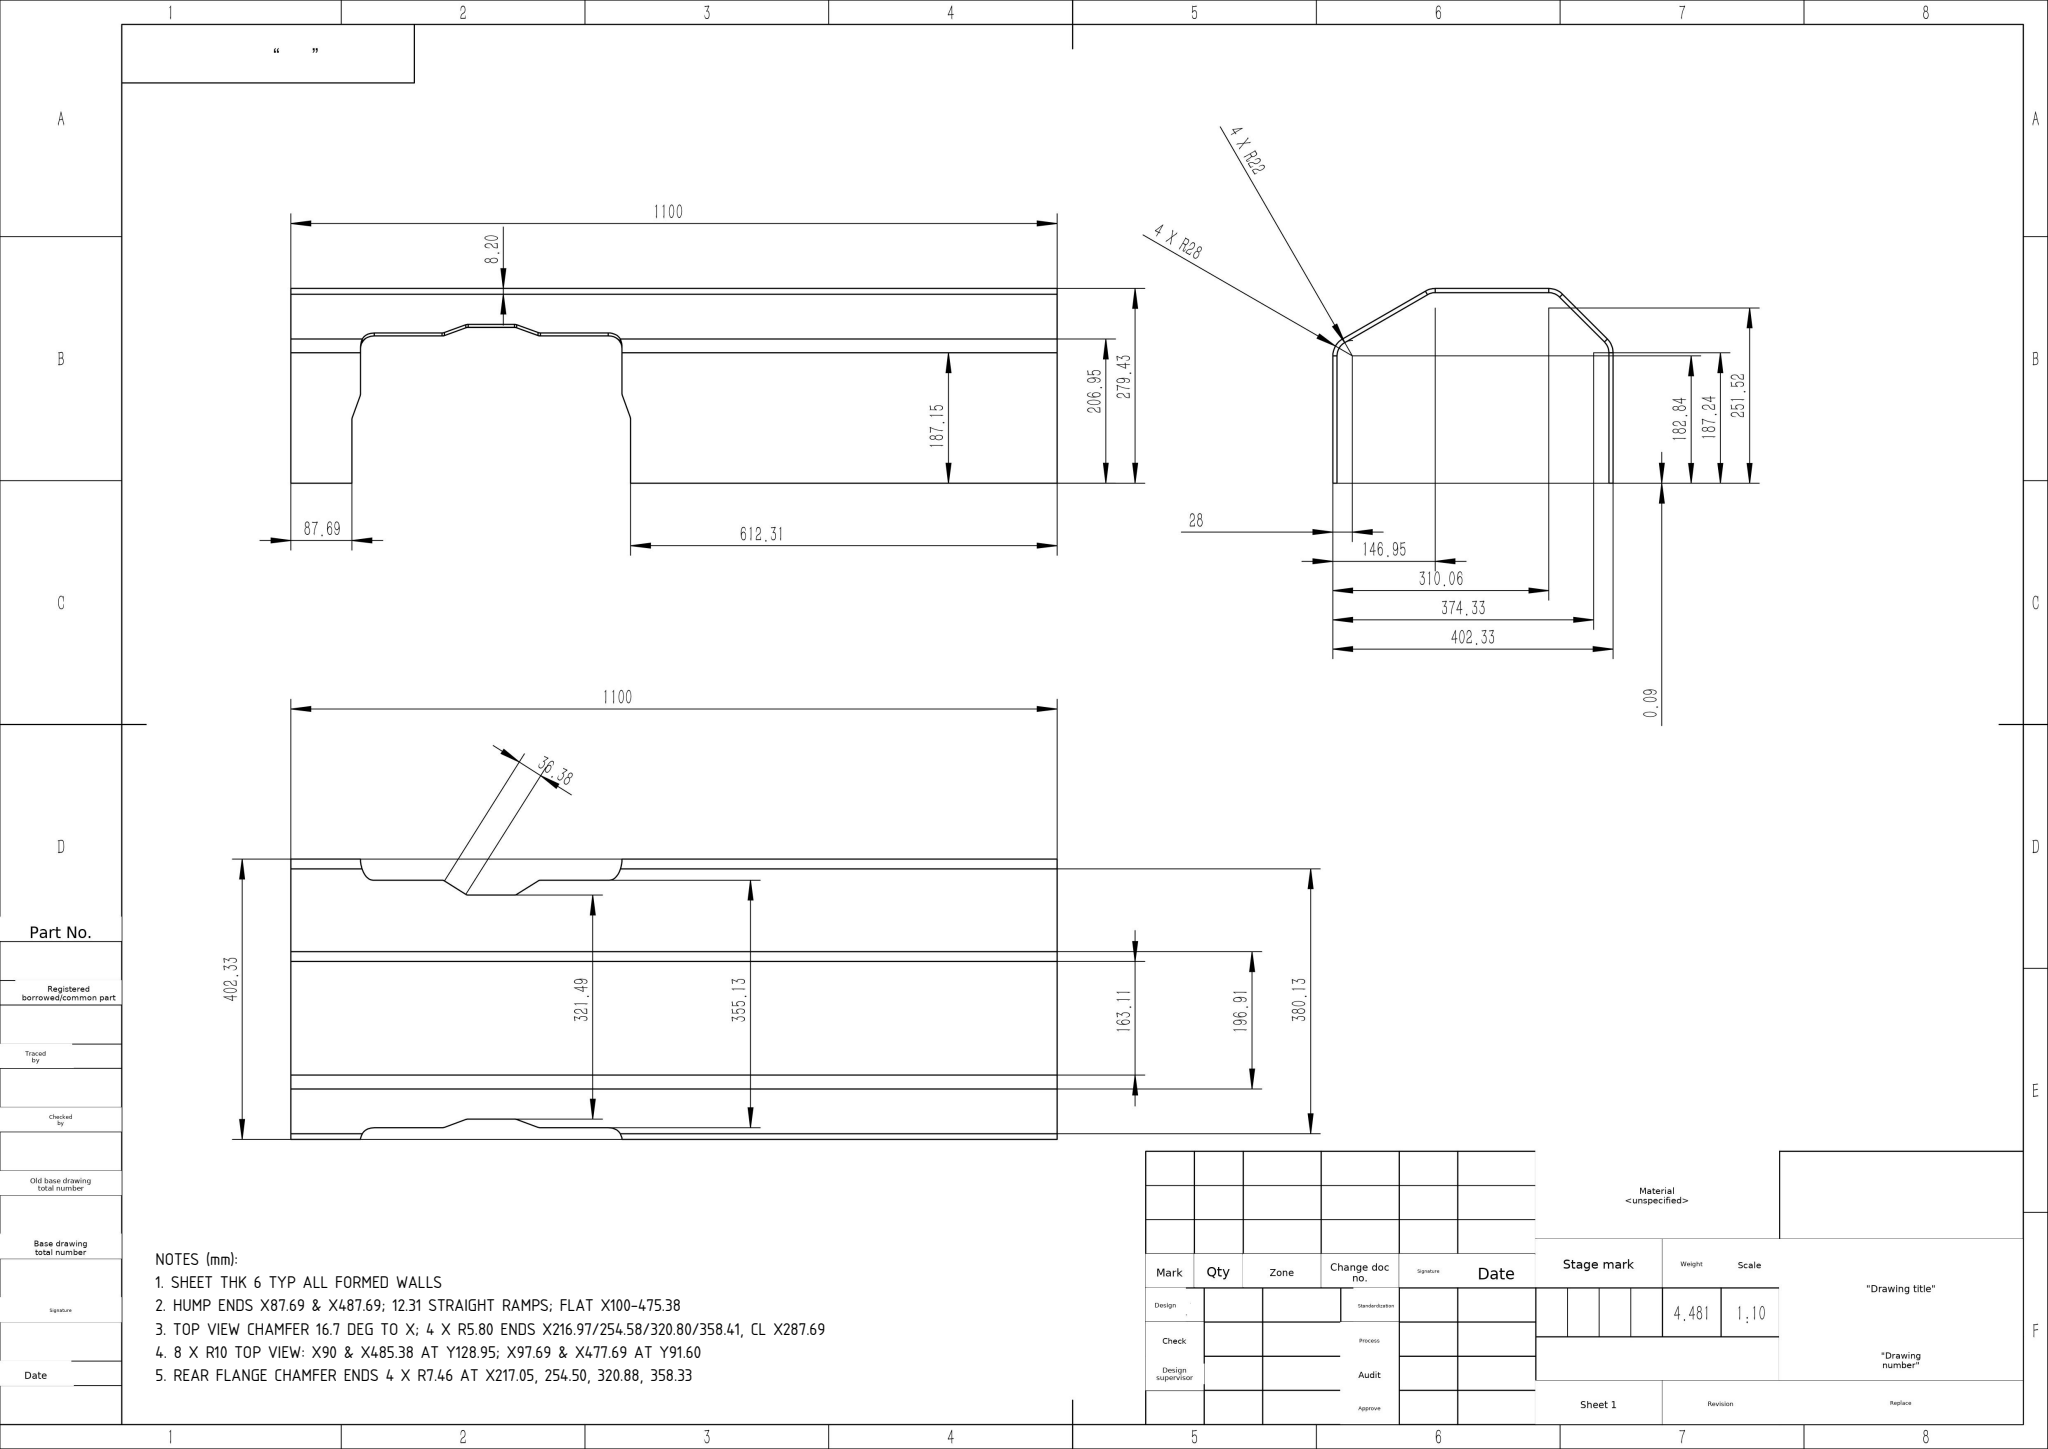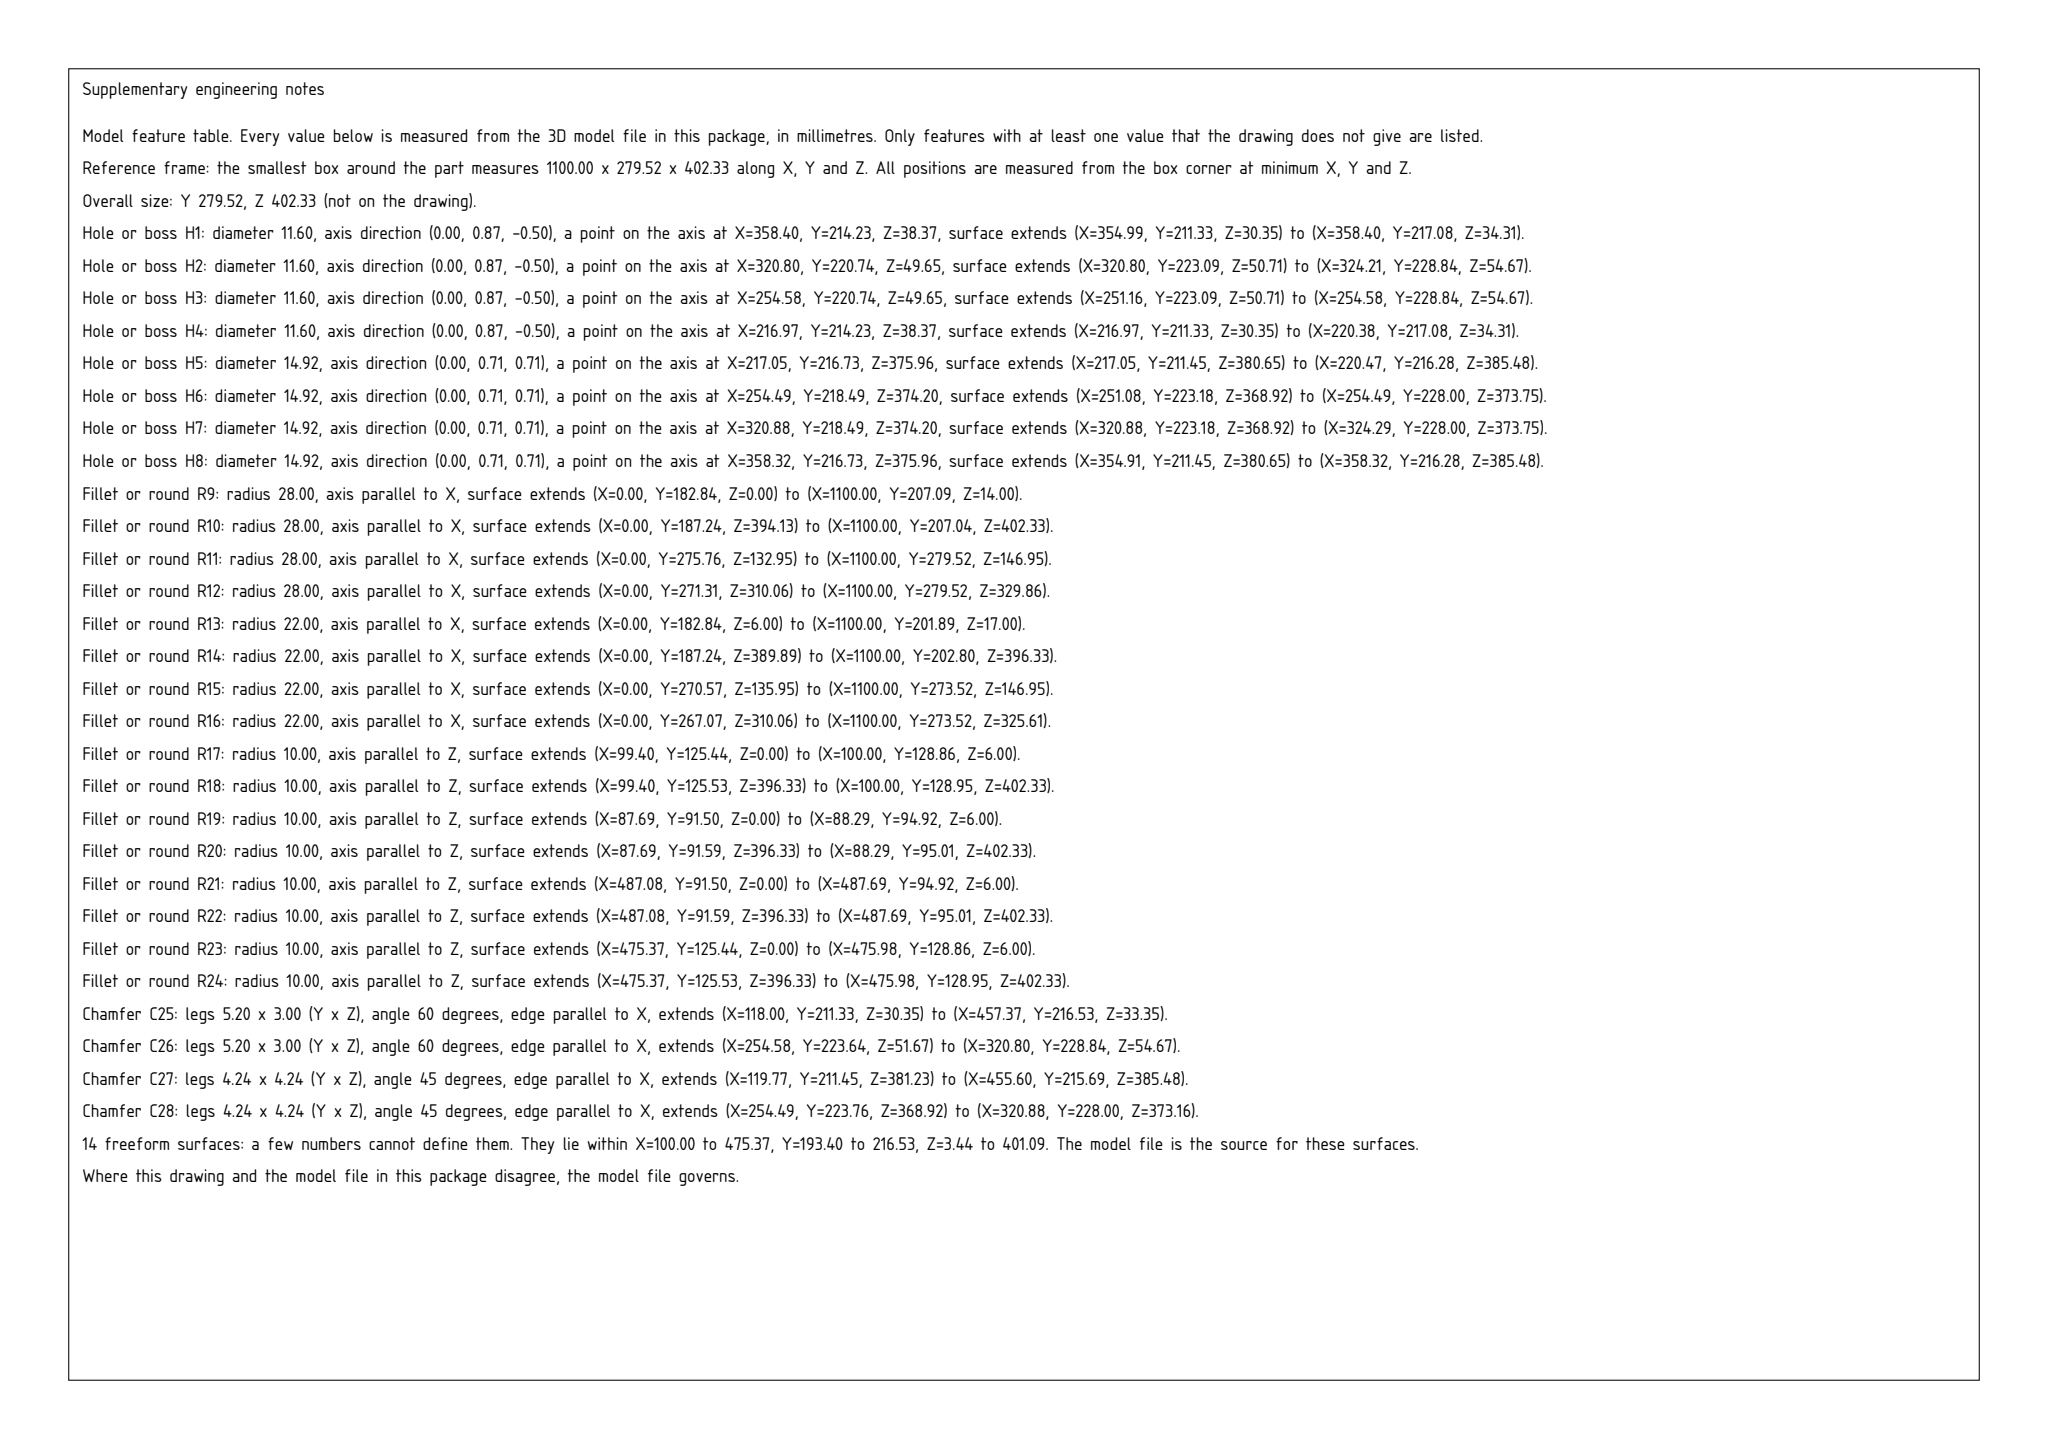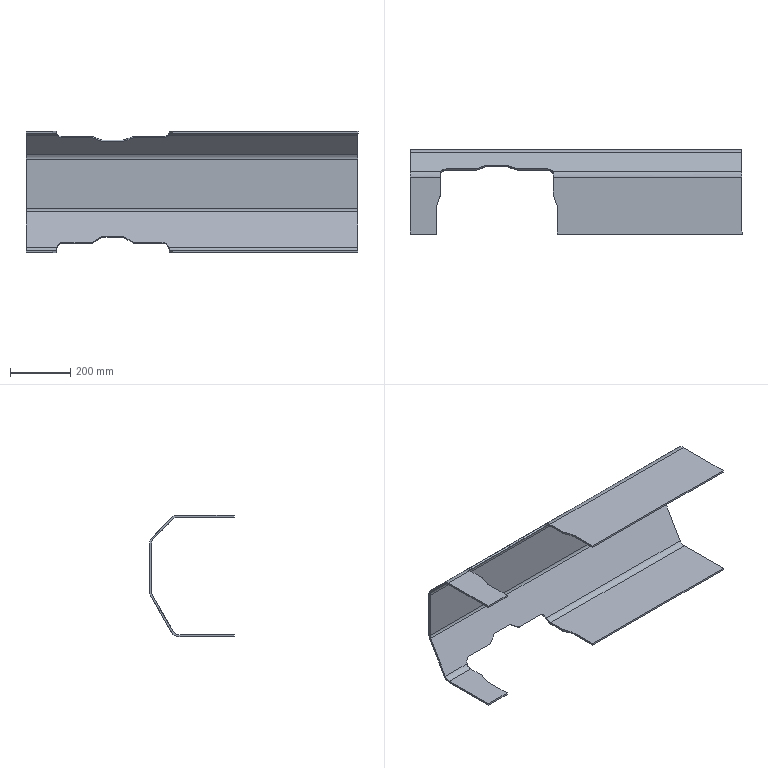Part | SolidWorks | mm | 1 solid | 104 faces | box 1100 x 279.52 x 402.33 mm | volume 4480851 mm3 | plane 62 | cylinder 28 | spline 14 | commonest cylinder face diameters 20 x8 44 x6 56 x6 11.603 x4 14.922 x4
Drawing notes:
SHEET THK 6 TYP ALL FORMED WALLS | from the solid: Face pairs Z0/Z6, Z396.33/Z402.33, Y273.52/Y279.52 all 6 apart; blend cyl len 5.75-6.0
HUMP ENDS X87.69 & X487.69; 12.31 STRAIGHT RAMPS; FLAT X100-475.38 | from the solid: x-normal planes at 87.69, 100.0, 475.38, 487.69 (none between); fillet_radii list empty
TOP VIEW CHAMFER 16.7 DEG TO X; 4 X R5.80 ENDS X216.97/254.58/320.80/358.41, CL X287.69 | from the solid: Dia 11.603 y-axis cyls at (216.97,38.37),(254.58,49.65),(320.80,49.65),(358.41,38.37); dz11.28/dx37.61=16.69 deg; sym about X287.69
8 X R10 TOP VIEW: X90 & X485.38 AT Y128.95; X97.69 & X477.69 AT Y91.60 | from the solid: Dia 20.0 z-axis cyls at (90,128.86/128.95),(97.69,91.51/91.6),(477.69,91.51/91.6),(485.38,128.86/128.95), len 6.0
REAR FLANGE CHAMFER ENDS 4 X R7.46 AT X217.05, 254.50, 320.88, 358.33 | from the solid: Dia 14.922 y-axis cyls at x=217.05/254.5/320.88/358.33, z=375.96/374.2, len 4.83